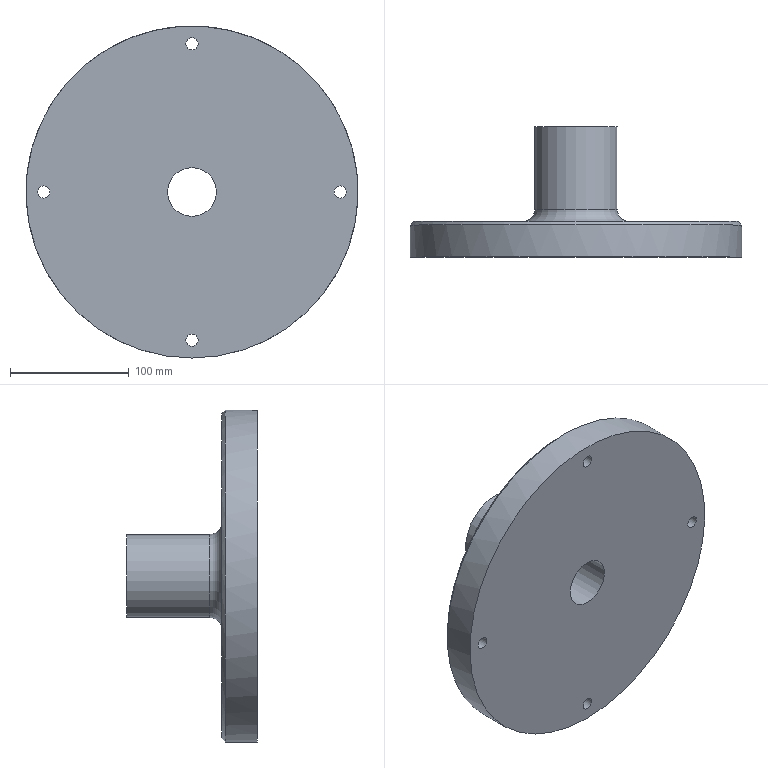Component | NX | SHUNK | 1 solid | 21 faces | volume 1989356 mm3 | cylinder 11 | plane 7 | cone 2 | torus 1 | commonest cylinder face diameters 10.2 x4 18.5 x4 280 x1 70 x1 41 x1